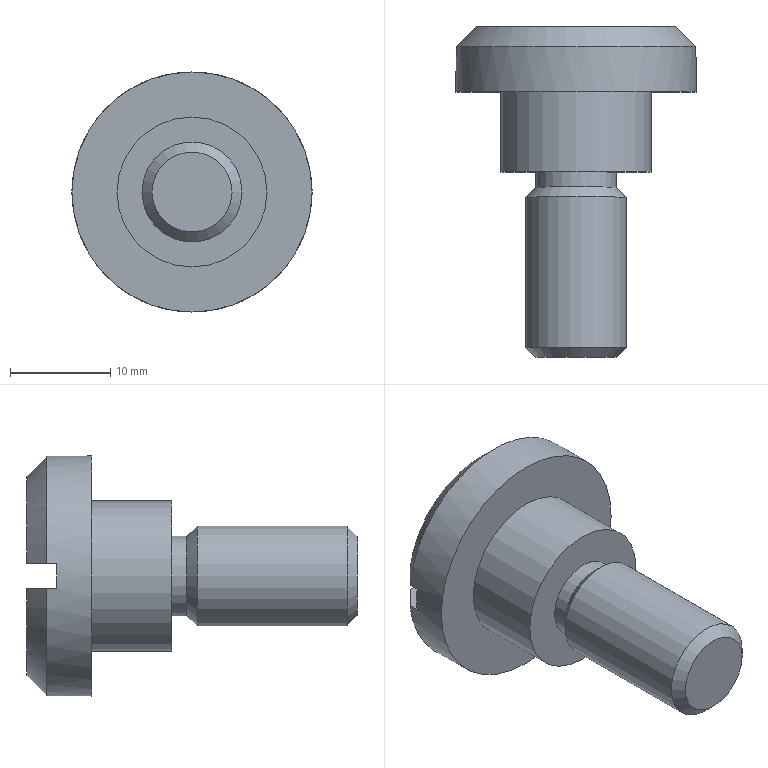Component | NX | BUSHING_SCREW | 1 solid | 16 faces | volume 5423 mm3 | plane 8 | cylinder 4 | cone 4 | commonest cylinder face diameters 10 x1 8 x1 15 x1 24 x1